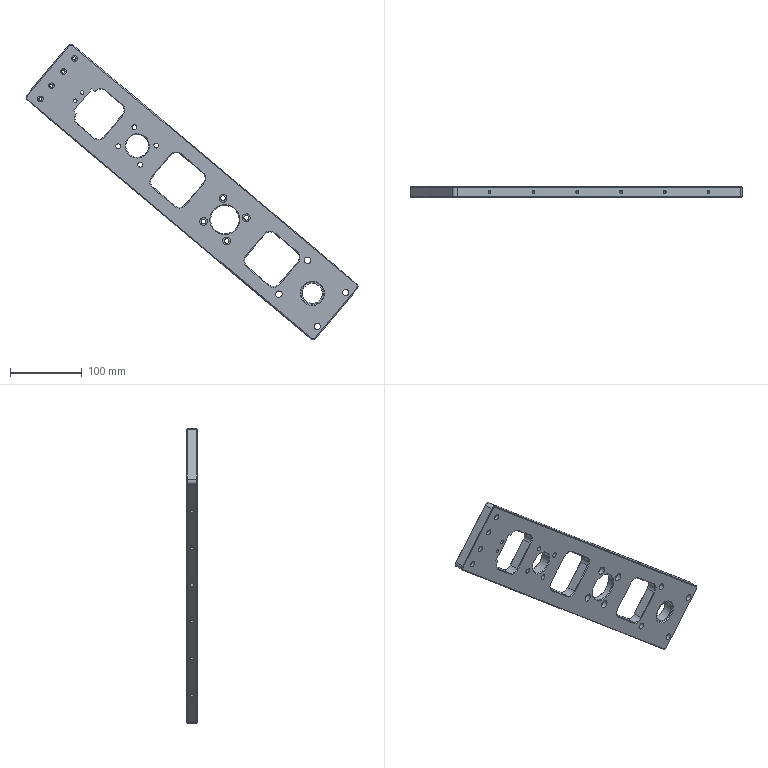Component | SolidWorks | 02GripperBasePlate-1 | 1 solid | 276 faces | box 464.22 x 15 x 412.47 mm | volume 565573 mm3 | cylinder 120 | cone 80 | plane 76 | commonest cylinder face diameters 5 x28 20 x12 3 x8 8 x8 15 x8 9 x8 6.8 x8 11 x8 | material Aviation Aluminum-7075
build123d program:
from build123d import *

# Parameters (mm, degrees)
SKETCH1_W                                           = 100
SKETCH1_H                                           = 408
BOSS_EXTRUDE1_DEPTH                                 = 15
CUT_EXTRUDE1_REACH                                  = 212.573
SKETCH2_R                                           = 16
SKETCH3_W                                           = 60
SKETCH3_H                                           = 60
CUT_EXTRUDE7_DEPTH                                  = 5
FILLET5_R                                           = 5
CUT_EXTRUDE6_REACH                                  = 212.276
SKETCH15_R                                          = 20
HOLE_SIZE_ACCORDING_TO_TYPE_2_OF_HEXAG_D            = 6.6
HOLE_SIZE_ACCORDING_TO_TYPE_2_OF_HEXAG_CBORE_D      = 11
HOLE_SIZE_ACCORDING_TO_TYPE_2_OF_HEXAG_CBORE_DEPTH  = 6.8
CIRPATTERN1_COUNT                                   = 4
CUT_EXTRUDE4_REACH                                  = 212.573
SKETCH8_W                                           = 60
SKETCH8_H                                           = 60
FILLET2_R                                           = 10
SKETCH10_W                                          = 100
SKETCH10_H                                          = 120
BOSS_EXTRUDE4_DEPTH                                 = 15
CUT_EXTRUDE5_REACH                                  = 330.178
SKETCH11_W                                          = 60
SKETCH11_H                                          = 50
FILLET3_R                                           = 10
FILLET4_R                                           = 5
M8_TAPPED_HOLE1_D                                   = 6.8
CHAMFER4_SIZE                                       = 1
CHAMFER6_SIZE                                       = 0.5
HOLE_SIZE_ACCORDING_TO_TYPE_3_OF_HEXAG_D            = 9
HOLE_SIZE_ACCORDING_TO_TYPE_3_OF_HEXAG_CBORE_D      = 15
HOLE_SIZE_ACCORDING_TO_TYPE_3_OF_HEXAG_CBORE_DEPTH  = 9
CHAMFER7_SIZE                                       = 1
CHAMFER8_SIZE                                       = 1
M3_TAPPED_HOLE1_D                                   = 2.5
LPATTERN1_COUNT                                     = 6
LPATTERN1_PITCH                                     = 80
SKETCH24_W                                          = 40
SKETCH24_H                                          = 40
CUT_EXTRUDE11_DEPTH                                 = 6
M6_TAPPED_HOLE2_D                                   = 5
M6_TAPPED_HOLE2_DEPTH                               = 15
M6_TAPPED_HOLE2_TIP                                 = 1.502
HOLE_SIZE_ACCORDING_TO_HEXAGON_SOCKET_H_D           = 4.5
HOLE_SIZE_ACCORDING_TO_HEXAGON_SOCKET_H_CBORE_D     = 8
HOLE_SIZE_ACCORDING_TO_HEXAGON_SOCKET_H_CBORE_DEPTH = 4.6
SKETCH27_R                                          = 4
CUT_EXTRUDE12_DEPTH                                 = 0.4
SKETCH28_R                                          = 1.5
CUT_EXTRUDE13_DEPTH                                 = 1.5
CHAMFER9_SIZE                                       = 0.2
BOSS_EXTRUDE5_START                                 = 13
SKETCH29_R                                          = 16
SKETCH29_R_2                                        = 14
BOSS_EXTRUDE5_DEPTH                                 = 13
CHAMFER11_SIZE                                      = 1


with BuildPart() as part:
    # Sketch1 → Boss-Extrude1 (new body)
    with BuildSketch(Plane.XY):
        Rectangle(SKETCH1_W, SKETCH1_H)
    extrude(amount=BOSS_EXTRUDE1_DEPTH)

    # Sketch2 → Cut-Extrude1 (cut, up to next)
    with BuildSketch(Plane.XY.offset(15), mode=Mode.PRIVATE) as cut_extrude1_sk1:
        with Locations((0, 160)):
            Circle(SKETCH2_R)
    cut_extrude1_tool1 = extrude(cut_extrude1_sk1.sketch, amount=-CUT_EXTRUDE1_REACH, mode=Mode.PRIVATE) & part.part
    # Sketch2 → Cut-Extrude1 (cut, up to next)
    with BuildSketch(Plane.XY.offset(15), mode=Mode.PRIVATE) as cut_extrude1_sk2:
        with Locations((0, -160)):
            Circle(SKETCH2_R)
    cut_extrude1_tool2 = extrude(cut_extrude1_sk2.sketch, amount=-CUT_EXTRUDE1_REACH, mode=Mode.PRIVATE) & part.part
    add(cut_extrude1_tool1.solids().sort_by_distance((0, 160, 15))[0], mode=Mode.SUBTRACT)
    add(cut_extrude1_tool2.solids().sort_by_distance((0, -160, 15))[0], mode=Mode.SUBTRACT)

    # Sketch3 → Cut-Extrude7 (cut)
    with BuildSketch(Plane(origin=(0, 0, 0), x_dir=(-1, 0, 0), z_dir=(0, 0, -1))):
        Rectangle(SKETCH3_W, SKETCH3_H)
    extrude(amount=-CUT_EXTRUDE7_DEPTH, mode=Mode.SUBTRACT)

    # Fillet5
    fillet5_edges = [part.edges().sort_by_distance(p)[0] for p in [
        (30, -30, 2.5),
        (30, 30, 2.5),
        (-30, 30, 2.5),
        (-30, -30, 2.5),
    ]]
    fillet(fillet5_edges, radius=FILLET5_R)

    # Sketch15 → Cut-Extrude6 (cut, up to next)
    with BuildSketch(Plane(origin=(0, 0, 5), x_dir=(-1, 0, 0), z_dir=(0, 0, -1)), mode=Mode.PRIVATE) as cut_extrude6_sk1:
        Circle(SKETCH15_R)
    cut_extrude6_tool1 = extrude(cut_extrude6_sk1.sketch, amount=-CUT_EXTRUDE6_REACH, mode=Mode.PRIVATE) & part.part
    add(cut_extrude6_tool1.solids().sort_by_distance((0, 0, 5))[0], mode=Mode.SUBTRACT)

    # Hole Size _According to_ Type 2 of Hexag (through all)
    with Locations(Plane(origin=(21.213, -21.213, 15), x_dir=(1, 0, 0), z_dir=(0, 0, 1))):
        with Locations((0, 0)):
            hole_size_according_to_type_2_of_hexag = CounterBoreHole(HOLE_SIZE_ACCORDING_TO_TYPE_2_OF_HEXAG_D / 2, HOLE_SIZE_ACCORDING_TO_TYPE_2_OF_HEXAG_CBORE_D / 2, HOLE_SIZE_ACCORDING_TO_TYPE_2_OF_HEXAG_CBORE_DEPTH)

    # CirPattern1: Hole Size _According to_ Type 2 of Hexag ×4 about axis
    cirpattern1_axis = Axis((0, 0, 0), (0, 0, 1))
    for i in range(1, CIRPATTERN1_COUNT):
        add(hole_size_according_to_type_2_of_hexag.rotate(cirpattern1_axis, i * 360 / CIRPATTERN1_COUNT), mode=Mode.SUBTRACT)

    # Sketch8 → Cut-Extrude4 (cut, up to next)
    with BuildSketch(Plane(origin=(0, 0, 0), x_dir=(-1, 0, 0), z_dir=(0, 0, -1)), mode=Mode.PRIVATE) as cut_extrude4_sk1:
        with Locations((0, 86)):
            Rectangle(SKETCH8_W, SKETCH8_H)
    cut_extrude4_tool1 = extrude(cut_extrude4_sk1.sketch, amount=-CUT_EXTRUDE4_REACH, mode=Mode.PRIVATE) & part.part
    # Sketch8 → Cut-Extrude4 (cut, up to next)
    with BuildSketch(Plane(origin=(0, 0, 0), x_dir=(-1, 0, 0), z_dir=(0, 0, -1)), mode=Mode.PRIVATE) as cut_extrude4_sk2:
        with Locations((0, -86)):
            Rectangle(SKETCH8_W, SKETCH8_H)
    cut_extrude4_tool2 = extrude(cut_extrude4_sk2.sketch, amount=-CUT_EXTRUDE4_REACH, mode=Mode.PRIVATE) & part.part
    add(cut_extrude4_tool1.solids().sort_by_distance((0, 86, 0))[0], mode=Mode.SUBTRACT)
    add(cut_extrude4_tool2.solids().sort_by_distance((0, -86, 0))[0], mode=Mode.SUBTRACT)

    # Fillet2
    fillet2_edges = [part.edges().sort_by_distance(p)[0] for p in [
        (30, 56, 7.5),
        (30, 116, 7.5),
        (-30, 116, 7.5),
        (-30, 56, 7.5),
        (30, -116, 7.5),
        (30, -56, 7.5),
        (-30, -56, 7.5),
        (-30, -116, 7.5),
    ]]
    fillet(fillet2_edges, radius=FILLET2_R)

    # Sketch10 → Boss-Extrude4 (add)
    with BuildSketch(Plane(origin=(0, 0, 0), x_dir=(-1, 0, 0), z_dir=(0, 0, -1))):
        with Locations((0, -264)):
            Rectangle(SKETCH10_W, SKETCH10_H)
    extrude(amount=-BOSS_EXTRUDE4_DEPTH)

    # Sketch11 → Cut-Extrude5 (cut, up to next)
    with BuildSketch(Plane(origin=(0, 0, 0), x_dir=(-1, 0, 0), z_dir=(0, 0, -1)), mode=Mode.PRIVATE) as cut_extrude5_sk1:
        with Locations((0, -229)):
            Rectangle(SKETCH11_W, SKETCH11_H)
    cut_extrude5_tool1 = extrude(cut_extrude5_sk1.sketch, amount=-CUT_EXTRUDE5_REACH, mode=Mode.PRIVATE) & part.part
    add(cut_extrude5_tool1.solids().sort_by_distance((0, -229, 0))[0], mode=Mode.SUBTRACT)

    # Fillet3
    fillet3_edges = [part.edges().sort_by_distance(p)[0] for p in [
        (30, -254, 7.5),
        (30, -204, 7.5),
        (-30, -204, 7.5),
        (-30, -254, 7.5),
    ]]
    fillet(fillet3_edges, radius=FILLET3_R)

    # Fillet4
    fillet4_edges = [part.edges().sort_by_distance(p)[0] for p in [
        (-50, -324, 7.5),
        (50, -324, 7.5),
        (-50, 204, 7.5),
        (50, 204, 7.5),
    ]]
    fillet(fillet4_edges, radius=FILLET4_R)

    # M8 Tapped Hole1 (through all)
    with Locations(Plane(origin=(-17.5, -140, 15), x_dir=(1, 0, 0), z_dir=(0, 0, 1))):
        with Locations((0, 0), (35, 0), (0, -40), (35, -40)):
            Hole(M8_TAPPED_HOLE1_D / 2)

    # Chamfer4
    chamfer4_edges = [part.edges().sort_by_distance(p)[0] for p in [
        (0, -116, 0),
        (0, -116, 15),
        (30, -86, 0),
        (30, -86, 15),
        (-30, -86, 0),
        (-30, -86, 15),
        (0, -56, 0),
        (0, -56, 15),
        (0, 56, 0),
        (0, 56, 15),
        (30, 86, 0),
        (30, 86, 15),
        (-30, 86, 0),
        (-30, 86, 15),
        (0, 116, 0),
        (0, 116, 15),
        (27.071, -113.071, 0),
        (27.071, -113.071, 15),
        (-27.071, -113.071, 0),
        (-27.071, -113.071, 15),
        (-27.071, -58.929, 0),
        (-27.071, -58.929, 15),
        (27.071, -58.929, 0),
        (27.071, -58.929, 15),
        (27.071, 58.929, 0),
        (27.071, 58.929, 15),
        (-27.071, 58.929, 0),
        (-27.071, 58.929, 15),
        (-27.071, 113.071, 0),
        (-27.071, 113.071, 15),
        (27.071, 113.071, 0),
        (27.071, 113.071, 15),
    ]]
    chamfer(chamfer4_edges, length=CHAMFER4_SIZE)

    # Chamfer6
    chamfer6_edges = [part.edges().sort_by_distance(p)[0] for p in [
        (-30, 0, 0),
        (0, -30, 0),
        (30, 0, 0),
        (0, 30, 0),
        (-28.536, -28.536, 0),
        (28.536, -28.536, 0),
        (28.536, 28.536, 0),
        (-28.536, 28.536, 0),
    ]]
    chamfer(chamfer6_edges, length=CHAMFER6_SIZE)

    # Hole Size _According to_ Type 3 of Hexag (through all)
    with Locations(Plane(origin=(31, 195, 0), x_dir=(-1, 0, 0), z_dir=(0, 0, -1))):
        with Locations((0, 0), (62, 0), (0, -70), (62, -70)):
            CounterBoreHole(HOLE_SIZE_ACCORDING_TO_TYPE_3_OF_HEXAG_D / 2, HOLE_SIZE_ACCORDING_TO_TYPE_3_OF_HEXAG_CBORE_D / 2, HOLE_SIZE_ACCORDING_TO_TYPE_3_OF_HEXAG_CBORE_DEPTH)

    # Chamfer7
    chamfer7_edges = [part.edges().sort_by_distance(p)[0] for p in [
        (0, -324, 15),
        (0, -324, 0),
        (-50, -60, 0),
        (0, 204, 0),
        (50, -60, 0),
        (48.536, 202.536, 0),
        (-48.536, 202.536, 0),
        (48.536, -322.536, 0),
        (-48.536, -322.536, 0),
        (-50, -60, 15),
        (50, -60, 15),
        (0, 204, 15),
        (48.536, 202.536, 15),
        (-48.536, 202.536, 15),
        (48.536, -322.536, 15),
        (-48.536, -322.536, 15),
    ]]
    chamfer(chamfer7_edges, length=CHAMFER7_SIZE)

    # Chamfer8
    chamfer8_edges = [part.edges().sort_by_distance(p)[0] for p in [
        (-30, -229, 0),
        (-30, -229, 15),
        (0, -254, 0),
        (0, -254, 15),
        (30, -229, 0),
        (30, -229, 15),
        (0, -204, 0),
        (0, -204, 15),
        (-27.071, -251.071, 0),
        (-27.071, -251.071, 15),
        (27.071, -251.071, 0),
        (27.071, -251.071, 15),
        (27.071, -206.929, 0),
        (27.071, -206.929, 15),
        (-27.071, -206.929, 0),
        (-27.071, -206.929, 15),
    ]]
    chamfer(chamfer8_edges, length=CHAMFER8_SIZE)

    # M3 Tapped Hole1 (through all)
    with Locations(Plane(origin=(37, -306, 0), x_dir=(-1, 0, 0), z_dir=(0, 0, -1))):
        with Locations((0, 0), (24, 0), (50, 0), (74, 0)):
            Hole(M3_TAPPED_HOLE1_D / 2)

    # Sketch23 → M6 Tapped Hole1 (revolve, cut)
    with BuildSketch(Plane(origin=(-50, 140, 7.5), x_dir=(0, 0, 1), z_dir=(0, 1, 0))):
        Polygon((0, 0), (0, 16.502), (2.5, 15), (2.5, 0), align=None)
    m6_tapped_hole1 = revolve(axis=Axis((-56.35, 140, 7.5), (1, 0, 0)), mode=Mode.SUBTRACT)

    # LPattern1: M6 Tapped Hole1 ×6
    with Locations(*[(0, -i * LPATTERN1_PITCH, 0) for i in range(1, LPATTERN1_COUNT)]):
        add(m6_tapped_hole1, mode=Mode.SUBTRACT)

    # Mirror1: M6 Tapped Hole1 across plane
    add(m6_tapped_hole1.mirror(Plane(origin=(0, 0, 0), x_dir=(0, 0, 1), z_dir=(1, 0, 0))), mode=Mode.SUBTRACT)

    # Mirror1 copy 1 sketch → Mirror1 copy 1 (revolve, cut)
    with BuildSketch(Plane(origin=(50, 60, 7.5), x_dir=(0, 0, 1), z_dir=(0, 1, 0))):
        Polygon((0, 0), (0, -16.502), (2.5, -15), (2.5, 0), align=None)
    revolve(axis=Axis((56.35, 60, 7.5), (1, 0, 0)), mode=Mode.SUBTRACT)

    # Mirror1 copy 2 sketch → Mirror1 copy 2 (revolve, cut)
    with BuildSketch(Plane(origin=(50, -20, 7.5), x_dir=(0, 0, 1), z_dir=(0, 1, 0))):
        Polygon((0, 0), (0, -16.502), (2.5, -15), (2.5, 0), align=None)
    revolve(axis=Axis((56.35, -20, 7.5), (1, 0, 0)), mode=Mode.SUBTRACT)

    # Mirror1 copy 3 sketch → Mirror1 copy 3 (revolve, cut)
    with BuildSketch(Plane(origin=(50, -100, 7.5), x_dir=(0, 0, 1), z_dir=(0, 1, 0))):
        Polygon((0, 0), (0, -16.502), (2.5, -15), (2.5, 0), align=None)
    revolve(axis=Axis((56.35, -100, 7.5), (1, 0, 0)), mode=Mode.SUBTRACT)

    # Mirror1 copy 4 sketch → Mirror1 copy 4 (revolve, cut)
    with BuildSketch(Plane(origin=(50, -180, 7.5), x_dir=(0, 0, 1), z_dir=(0, 1, 0))):
        Polygon((0, 0), (0, -16.502), (2.5, -15), (2.5, 0), align=None)
    revolve(axis=Axis((56.35, -180, 7.5), (1, 0, 0)), mode=Mode.SUBTRACT)

    # Mirror1 copy 5 sketch → Mirror1 copy 5 (revolve, cut)
    with BuildSketch(Plane(origin=(50, -260, 7.5), x_dir=(0, 0, 1), z_dir=(0, 1, 0))):
        Polygon((0, 0), (0, -16.502), (2.5, -15), (2.5, 0), align=None)
    revolve(axis=Axis((56.35, -260, 7.5), (1, 0, 0)), mode=Mode.SUBTRACT)

    # Sketch24 → Cut-Extrude11 (cut)
    with BuildSketch(Plane(origin=(0, -254, 0), x_dir=(1, 0, 0), z_dir=(0, 1, 0))):
        with Locations((0, -7.5)):
            Rectangle(SKETCH24_W, SKETCH24_H)
    extrude(amount=-CUT_EXTRUDE11_DEPTH, mode=Mode.SUBTRACT)

    # M6 Tapped Hole2
    with Locations(Plane(origin=(7.5, -267, 0), x_dir=(-1, 0, 0), z_dir=(0, 0, -1))):
        with Locations((0, 0), (15, 0)):
            Hole(M6_TAPPED_HOLE2_D / 2, depth=M6_TAPPED_HOLE2_DEPTH)
            with Locations((0, 0, -(M6_TAPPED_HOLE2_DEPTH + M6_TAPPED_HOLE2_TIP / 2))):  # 118° drill point
                Cone(0, M6_TAPPED_HOLE2_D / 2, M6_TAPPED_HOLE2_TIP, mode=Mode.SUBTRACT)

    # Hole Size_ according to_Hexagon Socket H (through all)
    with Locations(Plane(origin=(-37, -306, 15), x_dir=(1, 0, 0), z_dir=(0, 0, 1))):
        with Locations((0, 0), (24, 0), (50, 0), (74, 0)):
            CounterBoreHole(HOLE_SIZE_ACCORDING_TO_HEXAGON_SOCKET_H_D / 2, HOLE_SIZE_ACCORDING_TO_HEXAGON_SOCKET_H_CBORE_D / 2, HOLE_SIZE_ACCORDING_TO_HEXAGON_SOCKET_H_CBORE_DEPTH)

    # Sketch27 → Cut-Extrude12 (cut)
    with BuildSketch(Plane.XY.offset(10.4)):
        with Locations((37, -306)):
            Circle(SKETCH27_R)
        with Locations((13, -306)):
            Circle(SKETCH27_R)
        with Locations((-13, -306)):
            Circle(SKETCH27_R)
        with Locations((-37, -306)):
            Circle(SKETCH27_R)
    extrude(amount=-CUT_EXTRUDE12_DEPTH, mode=Mode.SUBTRACT)

    # Sketch28 → Cut-Extrude13 (cut)
    with BuildSketch(Plane(origin=(0, 0, 0), x_dir=(-1, 0, 0), z_dir=(0, 0, -1))):
        with Locations((-35, -318.34)):
            Circle(SKETCH28_R)
        with Locations((-15, -318.34)):
            Circle(SKETCH28_R)
        with Locations((15, -318.34)):
            Circle(SKETCH28_R)
        with Locations((35, -318.34)):
            Circle(SKETCH28_R)
    extrude(amount=-CUT_EXTRUDE13_DEPTH, mode=Mode.SUBTRACT)

    # Chamfer9
    chamfer9_edges = [part.edges().sort_by_distance(p)[0] for p in [
        (36.5, -318.34, 0),
        (16.5, -318.34, 0),
        (-13.5, -318.34, 0),
        (-33.5, -318.34, 0),
    ]]
    chamfer(chamfer9_edges, length=CHAMFER9_SIZE)

    # Sketch29 → Boss-Extrude5 (add)
    with BuildSketch(Plane.XY.offset(BOSS_EXTRUDE5_START)):
        with Locations((0, 160)):
            Circle(SKETCH29_R)
        with Locations(Location((0, 160, 0), (0, 0, 180))):
            Circle(SKETCH29_R_2, mode=Mode.SUBTRACT)
    extrude(amount=-BOSS_EXTRUDE5_DEPTH)

    # Chamfer11
    chamfer11_edges = [part.edges().sort_by_distance(p)[0] for p in [
        (-16, 160, 15),
        (-16, -160, 15),
        (-16, -160, 0),
        (20, 0, 15),
        (20, 0, 5),
        (14, 160, 0),
    ]]
    chamfer(chamfer11_edges, length=CHAMFER11_SIZE)


solid = part.part

# Placed as in the assembly
solid = solid.moved(Location((-144.488, 164.645, -264.11), (90, 0, -130.095)))